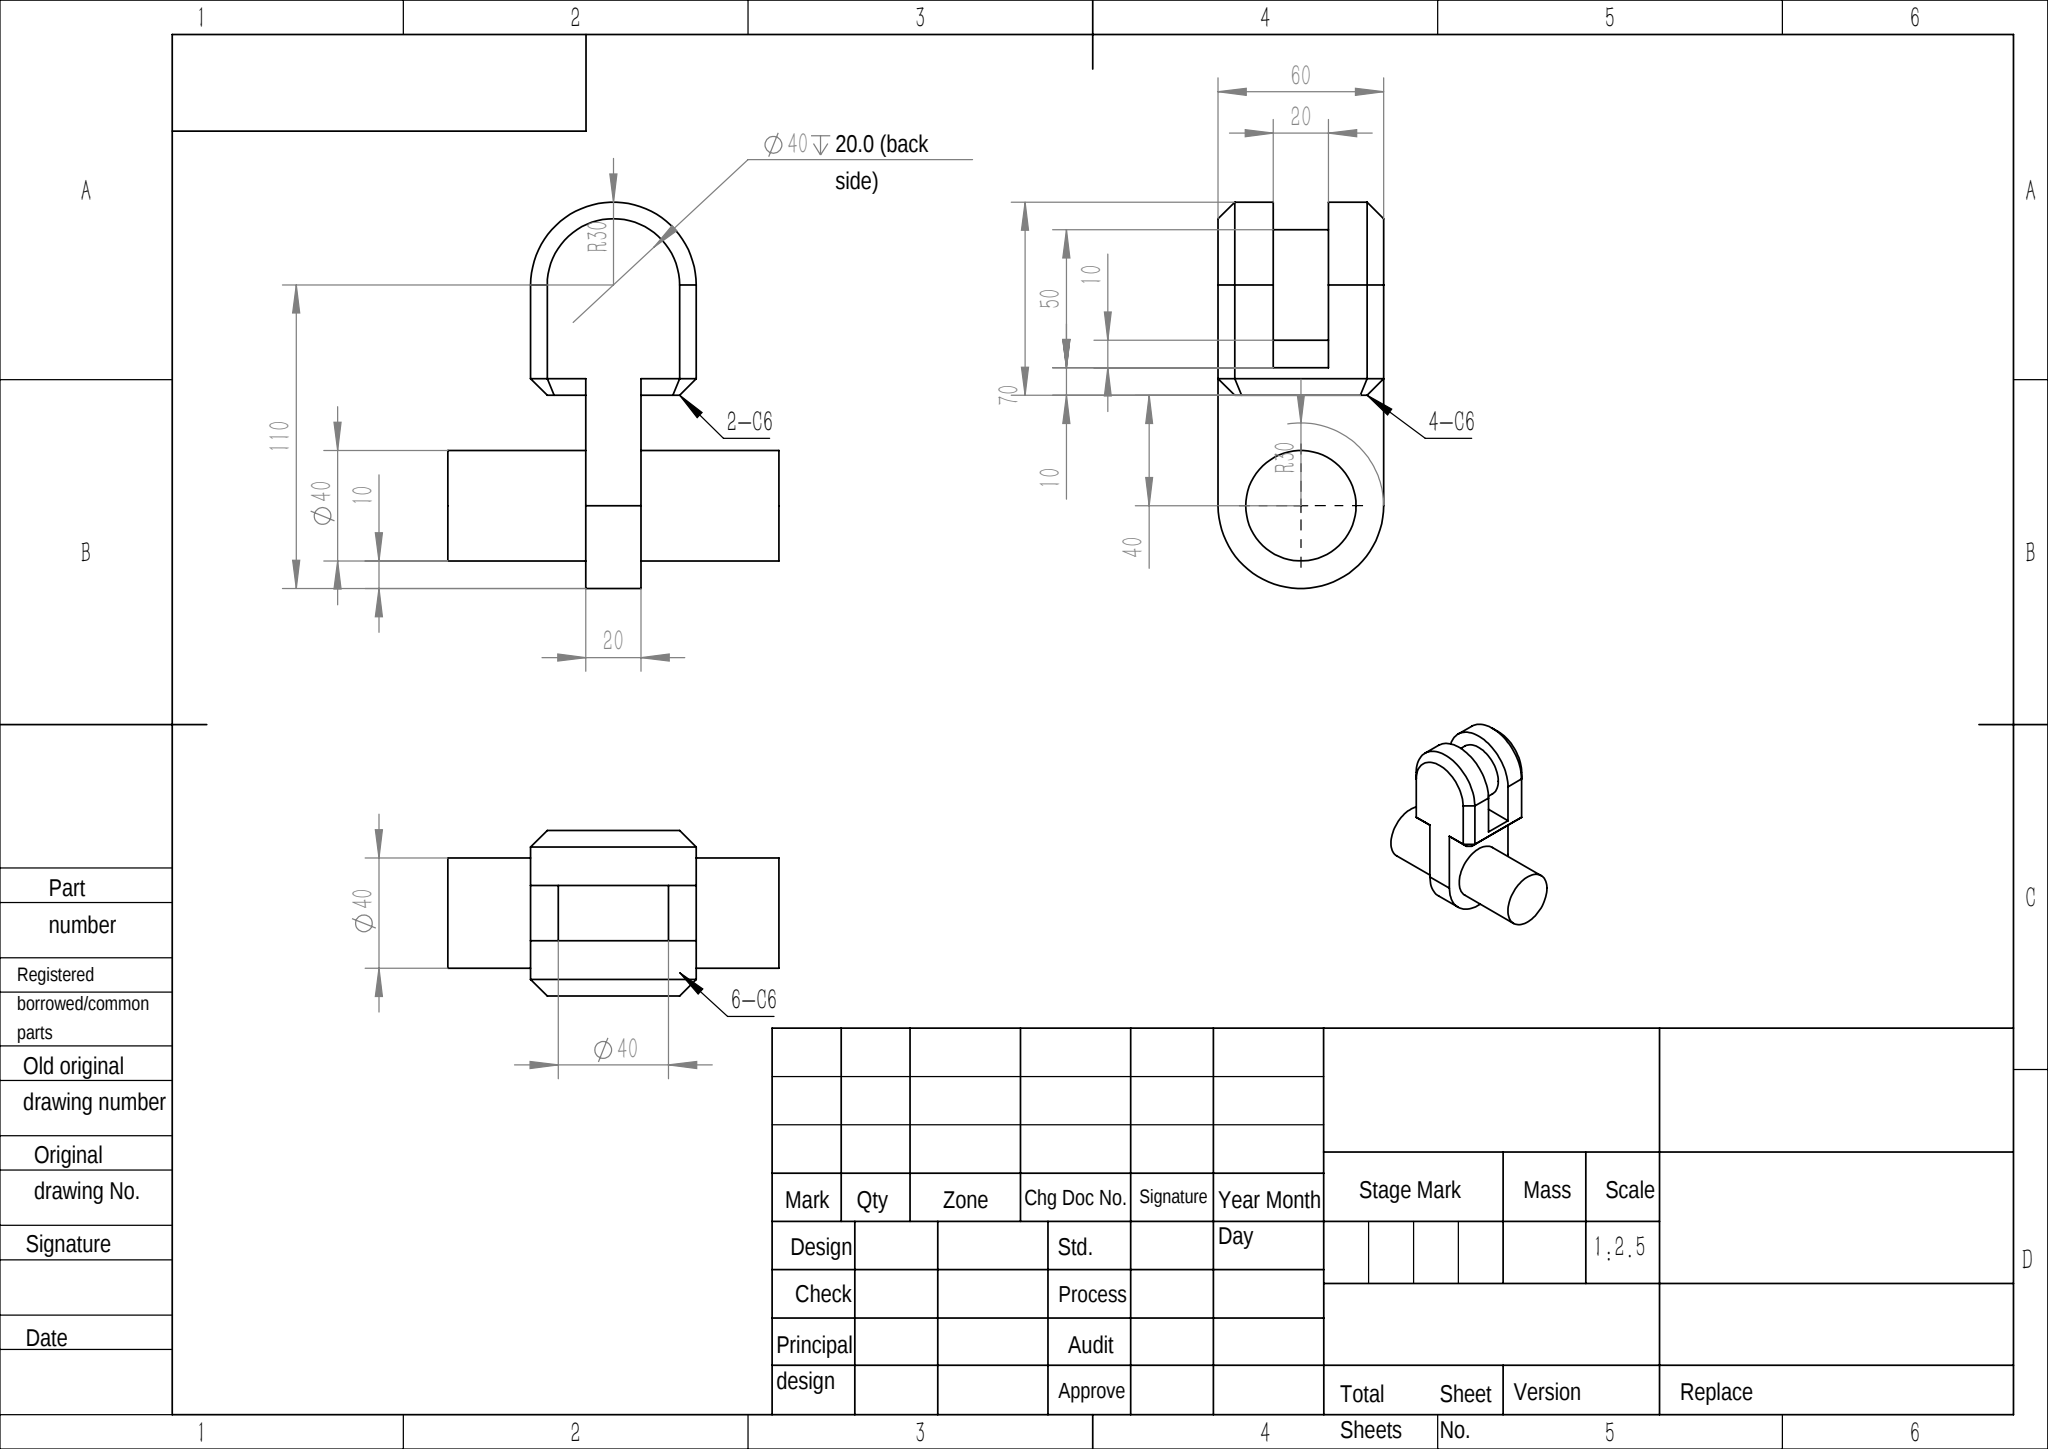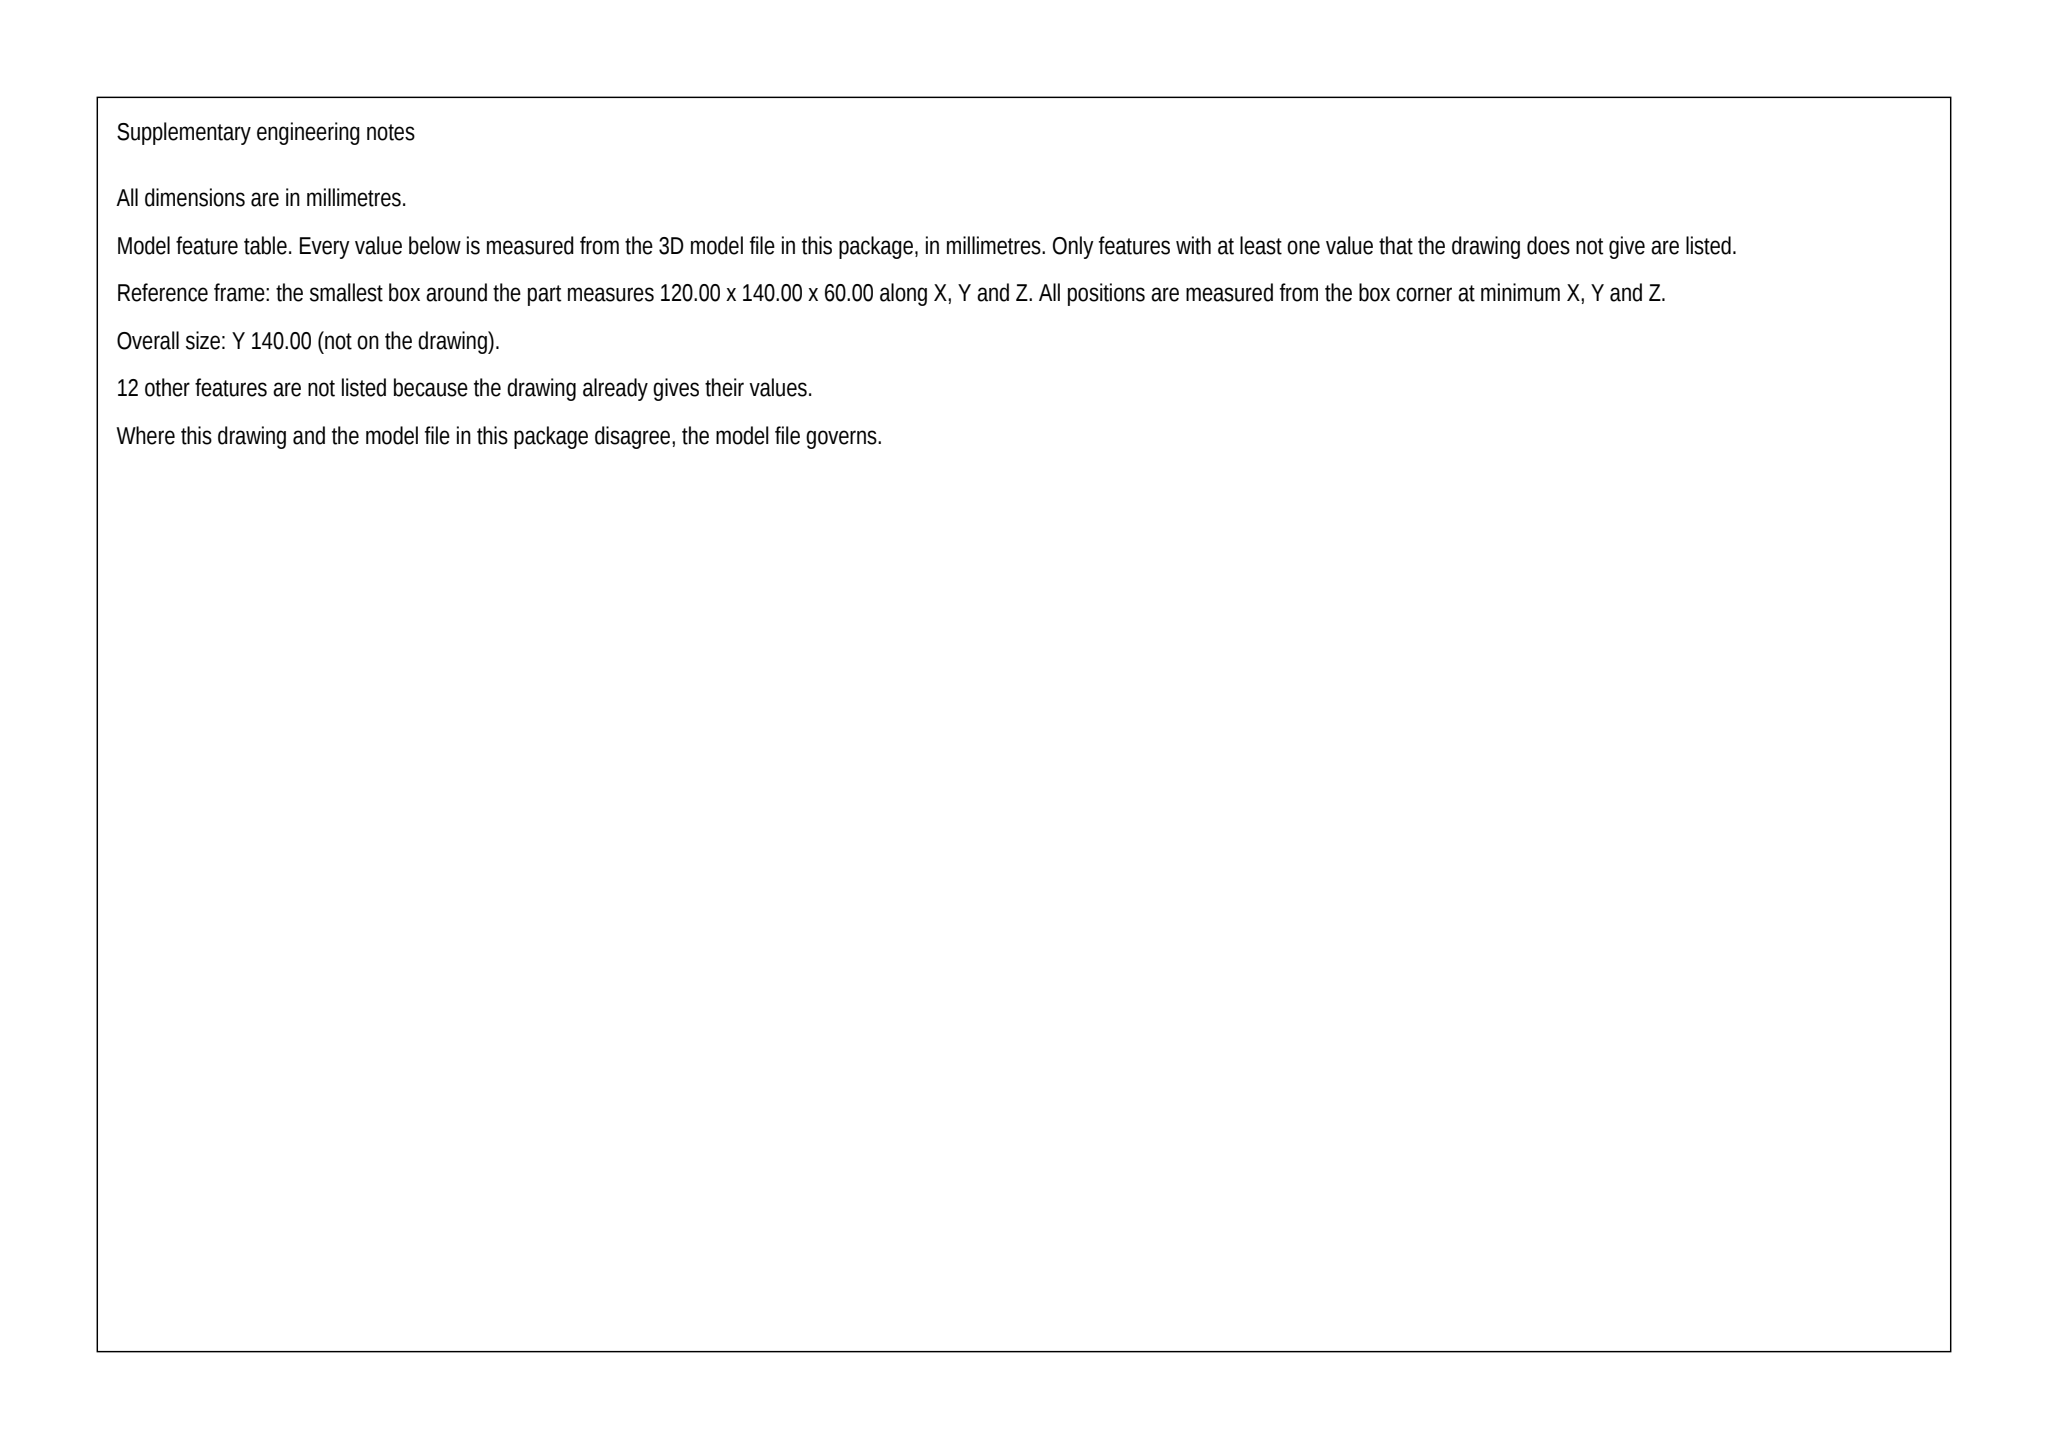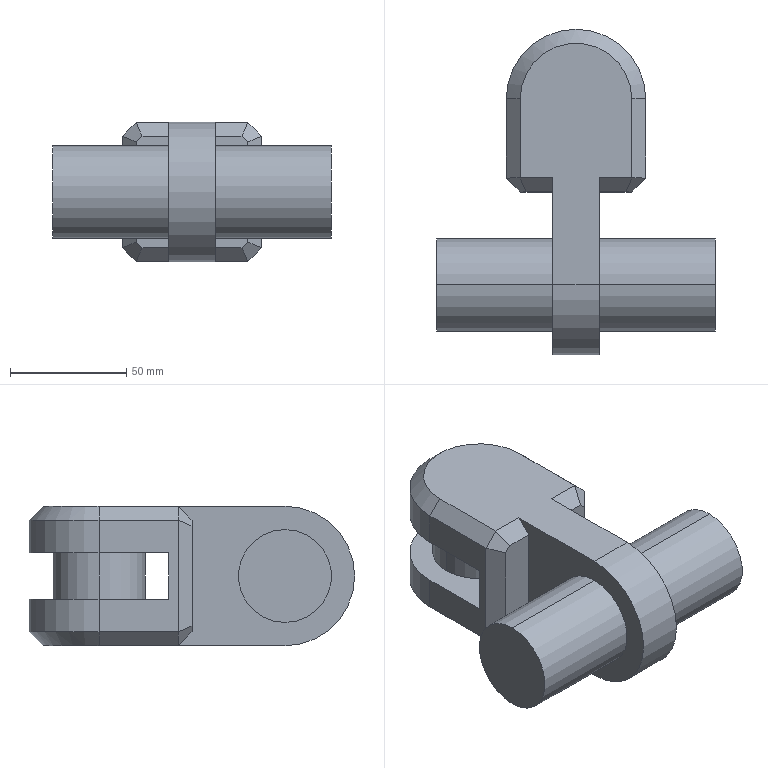Part | SolidWorks | mm | 1 solid | 38 faces | box 120 x 140 x 60 mm | volume 382464 mm3 | plane 27 | cylinder 9 | cone 2 | commonest cylinder face diameters 40 x6 60 x3
build123d program:
from build123d import *

# Parameters (mm, degrees)
BOSS_EXTRUDE1_DEPTH = 30
SKETCH2_R           = 20
BOSS_EXTRUDE2_DEPTH = 10
SKETCH3_R           = 20
CUT_EXTRUDE1_DEPTH  = 10
SKETCH4_R           = 20
BOSS_EXTRUDE3_DEPTH = 60
CHAMFER2_SIZE       = 6
CHAMFER1_SIZE       = 6


with BuildPart() as part:
    # Sketch1 → Boss-Extrude1 (new, symmetric)
    with BuildSketch(Plane.XY):
        with BuildLine():
            Line((-30, 0), (-30, -40))
            Line((-30, -40), (30, -40))
            Line((30, -40), (30, 0))
            ThreePointArc((30, 0), (0, 30), (-30, 0))
        make_face()
    extrude(amount=BOSS_EXTRUDE1_DEPTH, both=True)

    # Sketch2 → Boss-Extrude2 (add, symmetric)
    with BuildSketch(Plane(origin=(0, 0, 0), x_dir=(0, 0, -1), z_dir=(1, 0, 0))):
        with BuildLine():
            Line((-30, -80), (-30, -40))
            Line((-30, -40), (30, -40))
            Line((30, -40), (30, -80))
            ThreePointArc((30, -80), (0, -110), (-30, -80))
        make_face()
        with Locations((0, -80)):
            Circle(SKETCH2_R, mode=Mode.SUBTRACT)
    extrude(amount=BOSS_EXTRUDE2_DEPTH, both=True)

    # Sketch3 → Cut-Extrude1 (cut, symmetric)
    with BuildSketch(Plane.XY):
        with BuildLine():
            Line((-30, 0), (-30, -30))
            Line((-30, -30), (30, -30))
            Line((30, -30), (30, 0))
            ThreePointArc((30, 0), (0, 30), (-30, 0))
        make_face()
        Circle(SKETCH3_R, mode=Mode.SUBTRACT)
    extrude(amount=CUT_EXTRUDE1_DEPTH, both=True, mode=Mode.SUBTRACT)

    # Sketch4 → Boss-Extrude3 (add, symmetric)
    with BuildSketch(Plane(origin=(0, 0, 0), x_dir=(0, 0, -1), z_dir=(1, 0, 0))):
        with Locations((0, -80)):
            Circle(SKETCH4_R)
    extrude(amount=BOSS_EXTRUDE3_DEPTH, both=True)

    # Chamfer2
    chamfer2_edges = [part.edges().sort_by_distance(p)[0] for p in [
        (30, -20, -30),
        (-30, -20, -30),
        (0, 30, -30),
        (-30, -20, 30),
        (0, 30, 30),
        (30, -20, 30),
    ]]
    chamfer(chamfer2_edges, length=CHAMFER2_SIZE)

    # Chamfer1
    chamfer1_edges = [part.edges().sort_by_distance(p)[0] for p in [
        (-30, -40, 0),
        (30, -40, 0),
        (-17, -40, -30),
        (-17, -40, 30),
        (-27, -40, -27),
        (-27, -40, 27),
        (17, -40, -30),
        (17, -40, 30),
        (27, -40, 27),
        (27, -40, -27),
    ]]
    chamfer(chamfer1_edges, length=CHAMFER1_SIZE)


solid = part.part